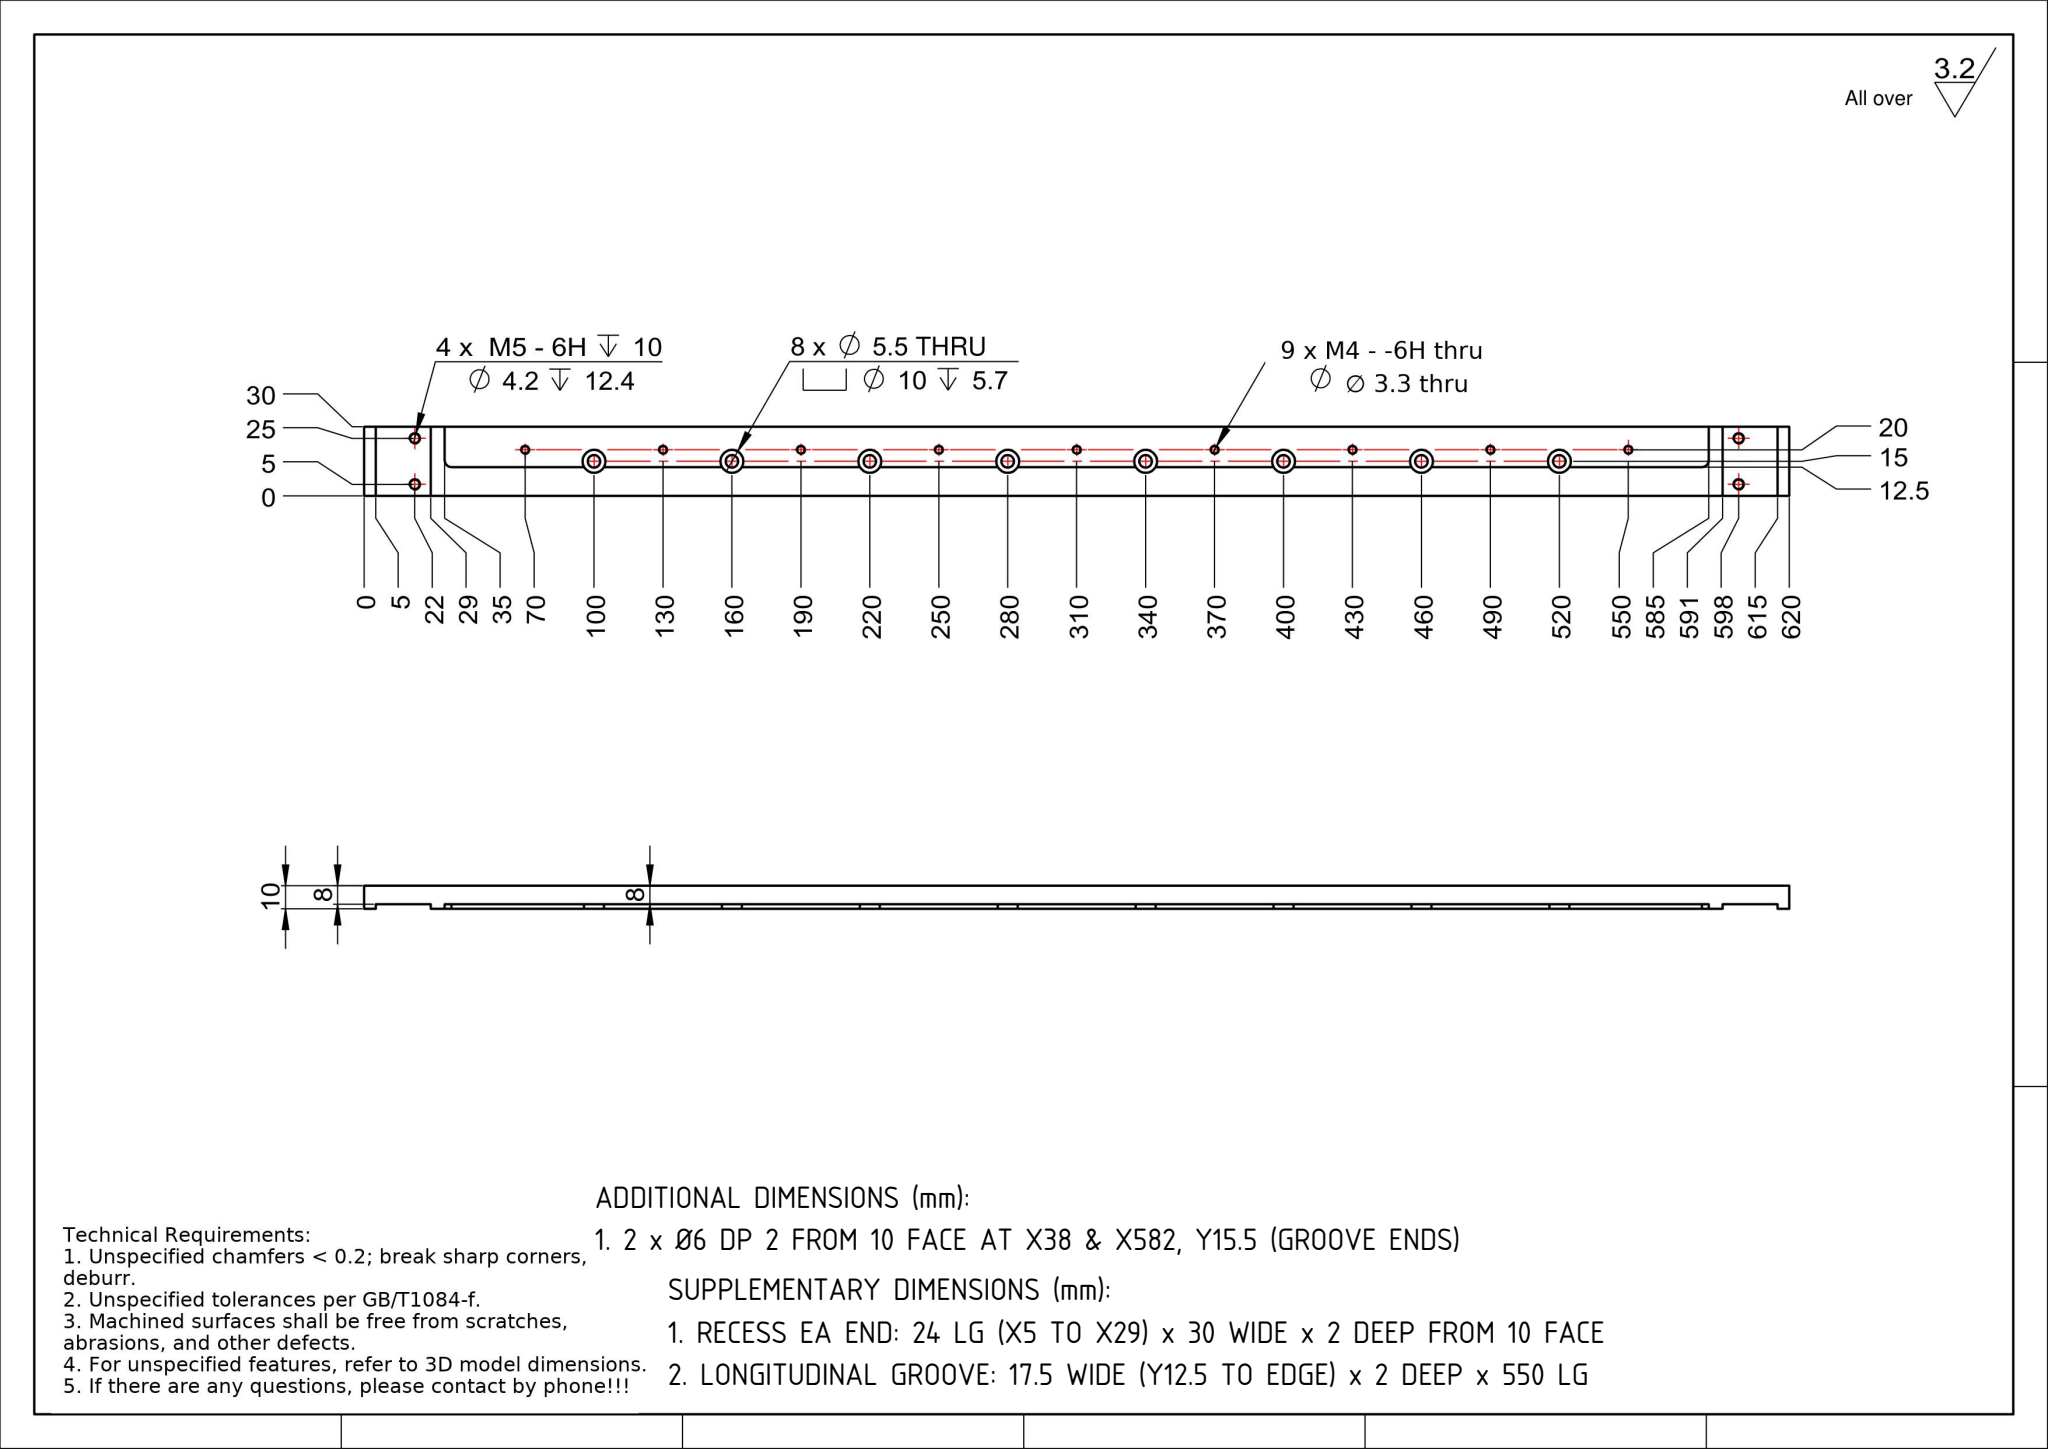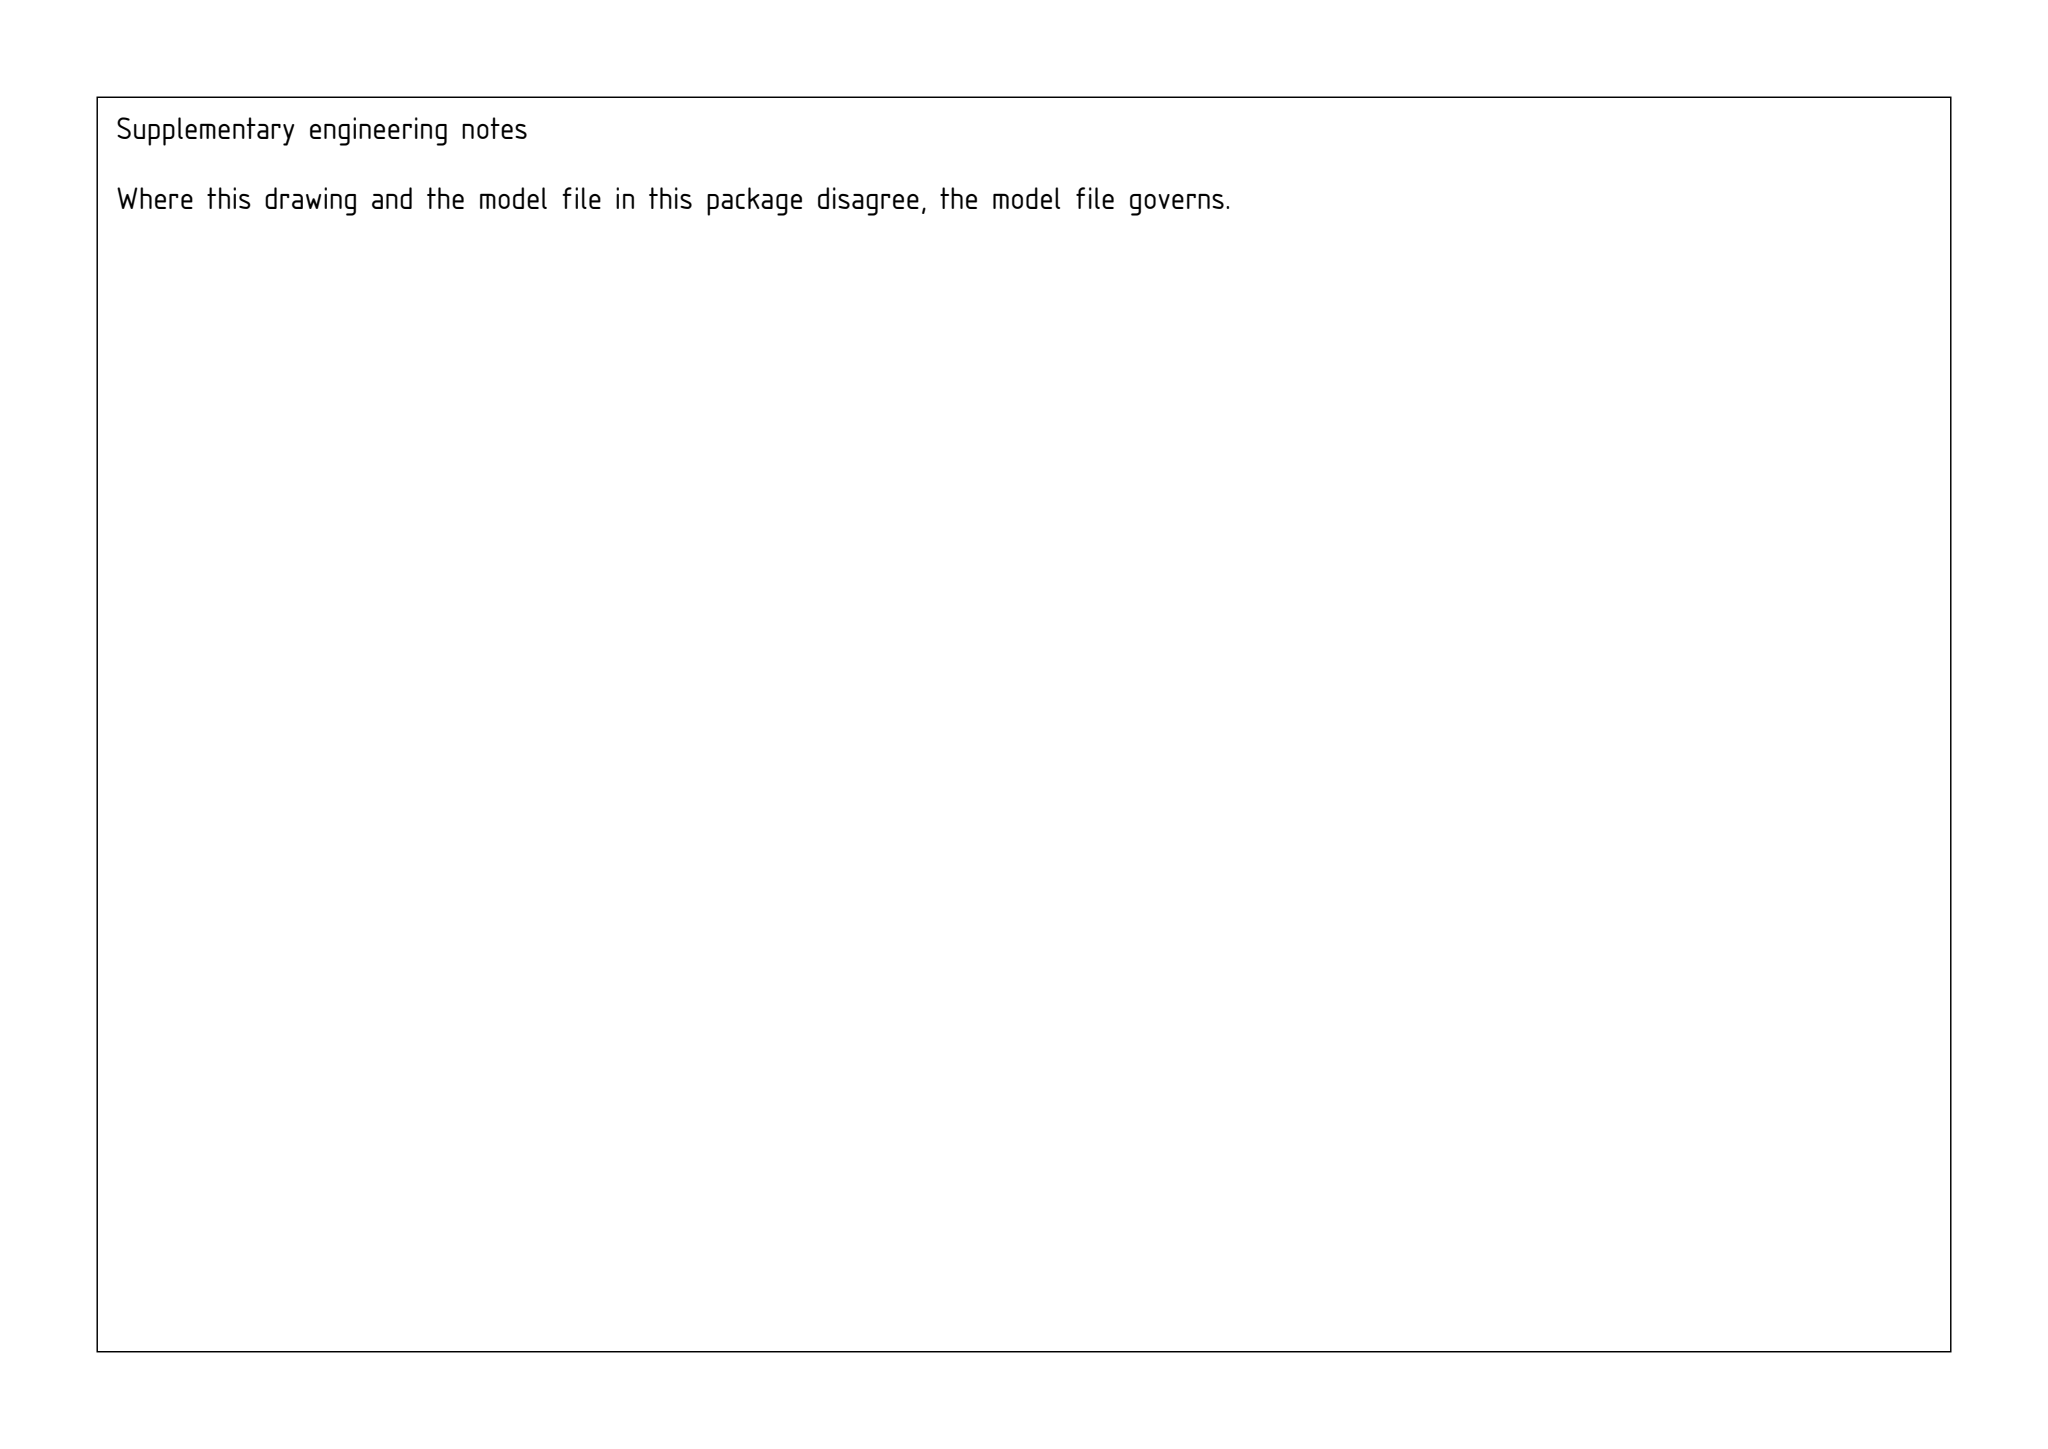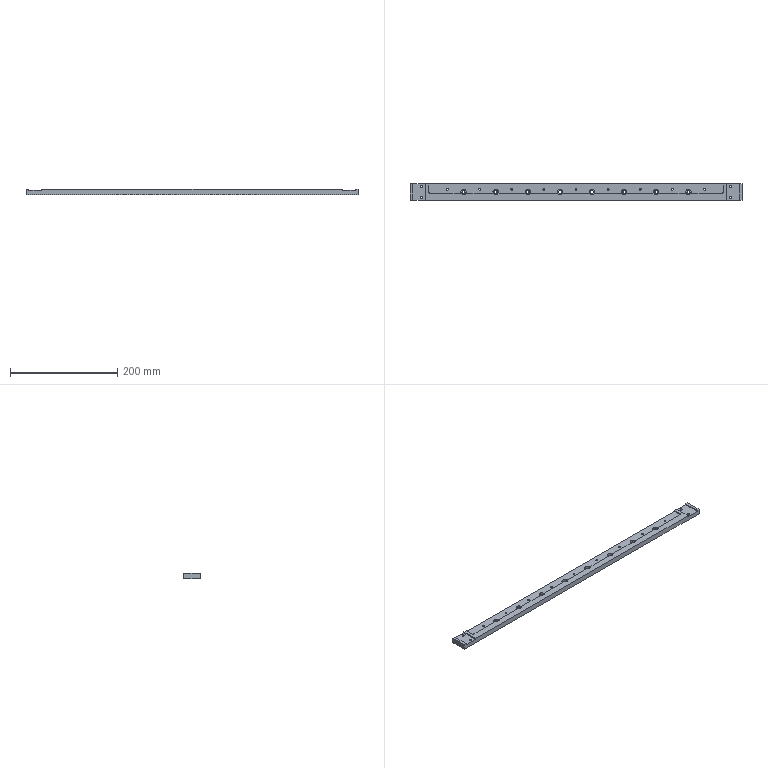Part | SolidWorks | mm | 1 solid | 94 faces | box 620 x 30 x 10 mm | volume 159431 mm3 | cylinder 60 | plane 34 | commonest cylinder face diameters 3.3 x18 5.5 x16 10 x16 4.2 x8 6 x2
build123d program:
from build123d import *

# Parameters (mm, degrees)
SKETCH1_W                                         = 620
SKETCH1_H                                         = 30
BOSS_EXTRUDE1_DEPTH                               = 5
SKETCH2_W                                         = 550
SKETCH2_H                                         = 17.5
CUT_EXTRUDE1_DEPTH                                = 2
M4_TAPPED_HOLE1_D                                 = 3.3
HOLE_SIZE_ACCORDING_TO_TYPE_1_OF_HEXA_D           = 5.5
HOLE_SIZE_ACCORDING_TO_TYPE_1_OF_HEXA_CBORE_D     = 10
HOLE_SIZE_ACCORDING_TO_TYPE_1_OF_HEXA_CBORE_DEPTH = 5.7
LPATTERN1_COUNT                                   = 9
LPATTERN1_PITCH                                   = 60
LPATTERN2_COUNT                                   = 8
LPATTERN2_PITCH                                   = 60
SKETCH7_W                                         = 24
SKETCH7_H                                         = 30
CUT_EXTRUDE2_DEPTH                                = 2
M5_TAPPED_HOLE1_D                                 = 4.2
M5_TAPPED_HOLE1_DEPTH                             = 12.4
M5_TAPPED_HOLE1_TIP                               = 1.262
FILLET1_R                                         = 3


with BuildPart() as part:
    # Sketch1 → Boss-Extrude1 (new, symmetric)
    with BuildSketch(Plane.XY):
        Rectangle(SKETCH1_W, SKETCH1_H)
    extrude(amount=BOSS_EXTRUDE1_DEPTH, both=True)

    # Sketch2 → Cut-Extrude1 (cut)
    with BuildSketch(Plane.XY.offset(5)):
        with Locations((0, 6.25)):
            Rectangle(SKETCH2_W, SKETCH2_H)
    extrude(amount=-CUT_EXTRUDE1_DEPTH, mode=Mode.SUBTRACT)

    # M4 Tapped Hole1 (through all)
    with Locations(Plane(origin=(0, 0, -5), x_dir=(-1, 0, 0), z_dir=(0, 0, -1))):
        with Locations((240, 5)):
            m4_tapped_hole1 = Hole(M4_TAPPED_HOLE1_D / 2)

    # Hole Size _ according to_ Type 1 of Hexa (through all)
    with Locations(Plane.XY.offset(5)):
        with Locations((210, 0)):
            hole_size_according_to_type_1_of_hexa = CounterBoreHole(HOLE_SIZE_ACCORDING_TO_TYPE_1_OF_HEXA_D / 2, HOLE_SIZE_ACCORDING_TO_TYPE_1_OF_HEXA_CBORE_D / 2, HOLE_SIZE_ACCORDING_TO_TYPE_1_OF_HEXA_CBORE_DEPTH)

    # LPattern1: M4 Tapped Hole1 ×9
    with Locations(*[(i * LPATTERN1_PITCH, 0, 0) for i in range(1, LPATTERN1_COUNT)]):
        add(m4_tapped_hole1, mode=Mode.SUBTRACT)

    # LPattern2: Hole Size _ according to_ Type 1 of Hexa ×8
    with Locations(*[(-i * LPATTERN2_PITCH, 0, 0) for i in range(1, LPATTERN2_COUNT)]):
        add(hole_size_according_to_type_1_of_hexa, mode=Mode.SUBTRACT)

    # Sketch7 → Cut-Extrude2 (cut)
    with BuildSketch(Plane.XY.offset(5)):
        with Locations((293, 0)):
            Rectangle(SKETCH7_W, SKETCH7_H)
        with Locations((-293, 0)):
            Rectangle(SKETCH7_W, SKETCH7_H)
    extrude(amount=-CUT_EXTRUDE2_DEPTH, mode=Mode.SUBTRACT)

    # M5 Tapped Hole1
    with Locations(Plane.XY.offset(3)):
        with Locations((288, 10), (288, -10), (-288, 10), (-288, -10)):
            Hole(M5_TAPPED_HOLE1_D / 2, depth=M5_TAPPED_HOLE1_DEPTH)
            with Locations((0, 0, -(M5_TAPPED_HOLE1_DEPTH + M5_TAPPED_HOLE1_TIP / 2))):  # 118° drill point
                Cone(0, M5_TAPPED_HOLE1_D / 2, M5_TAPPED_HOLE1_TIP, mode=Mode.SUBTRACT)

    # Fillet1
    fillet1_edges = [part.edges().sort_by_distance(p)[0] for p in [
        (-275, -2.5, 4),
        (275, -2.5, 4),
    ]]
    fillet(fillet1_edges, radius=FILLET1_R)


solid = part.part